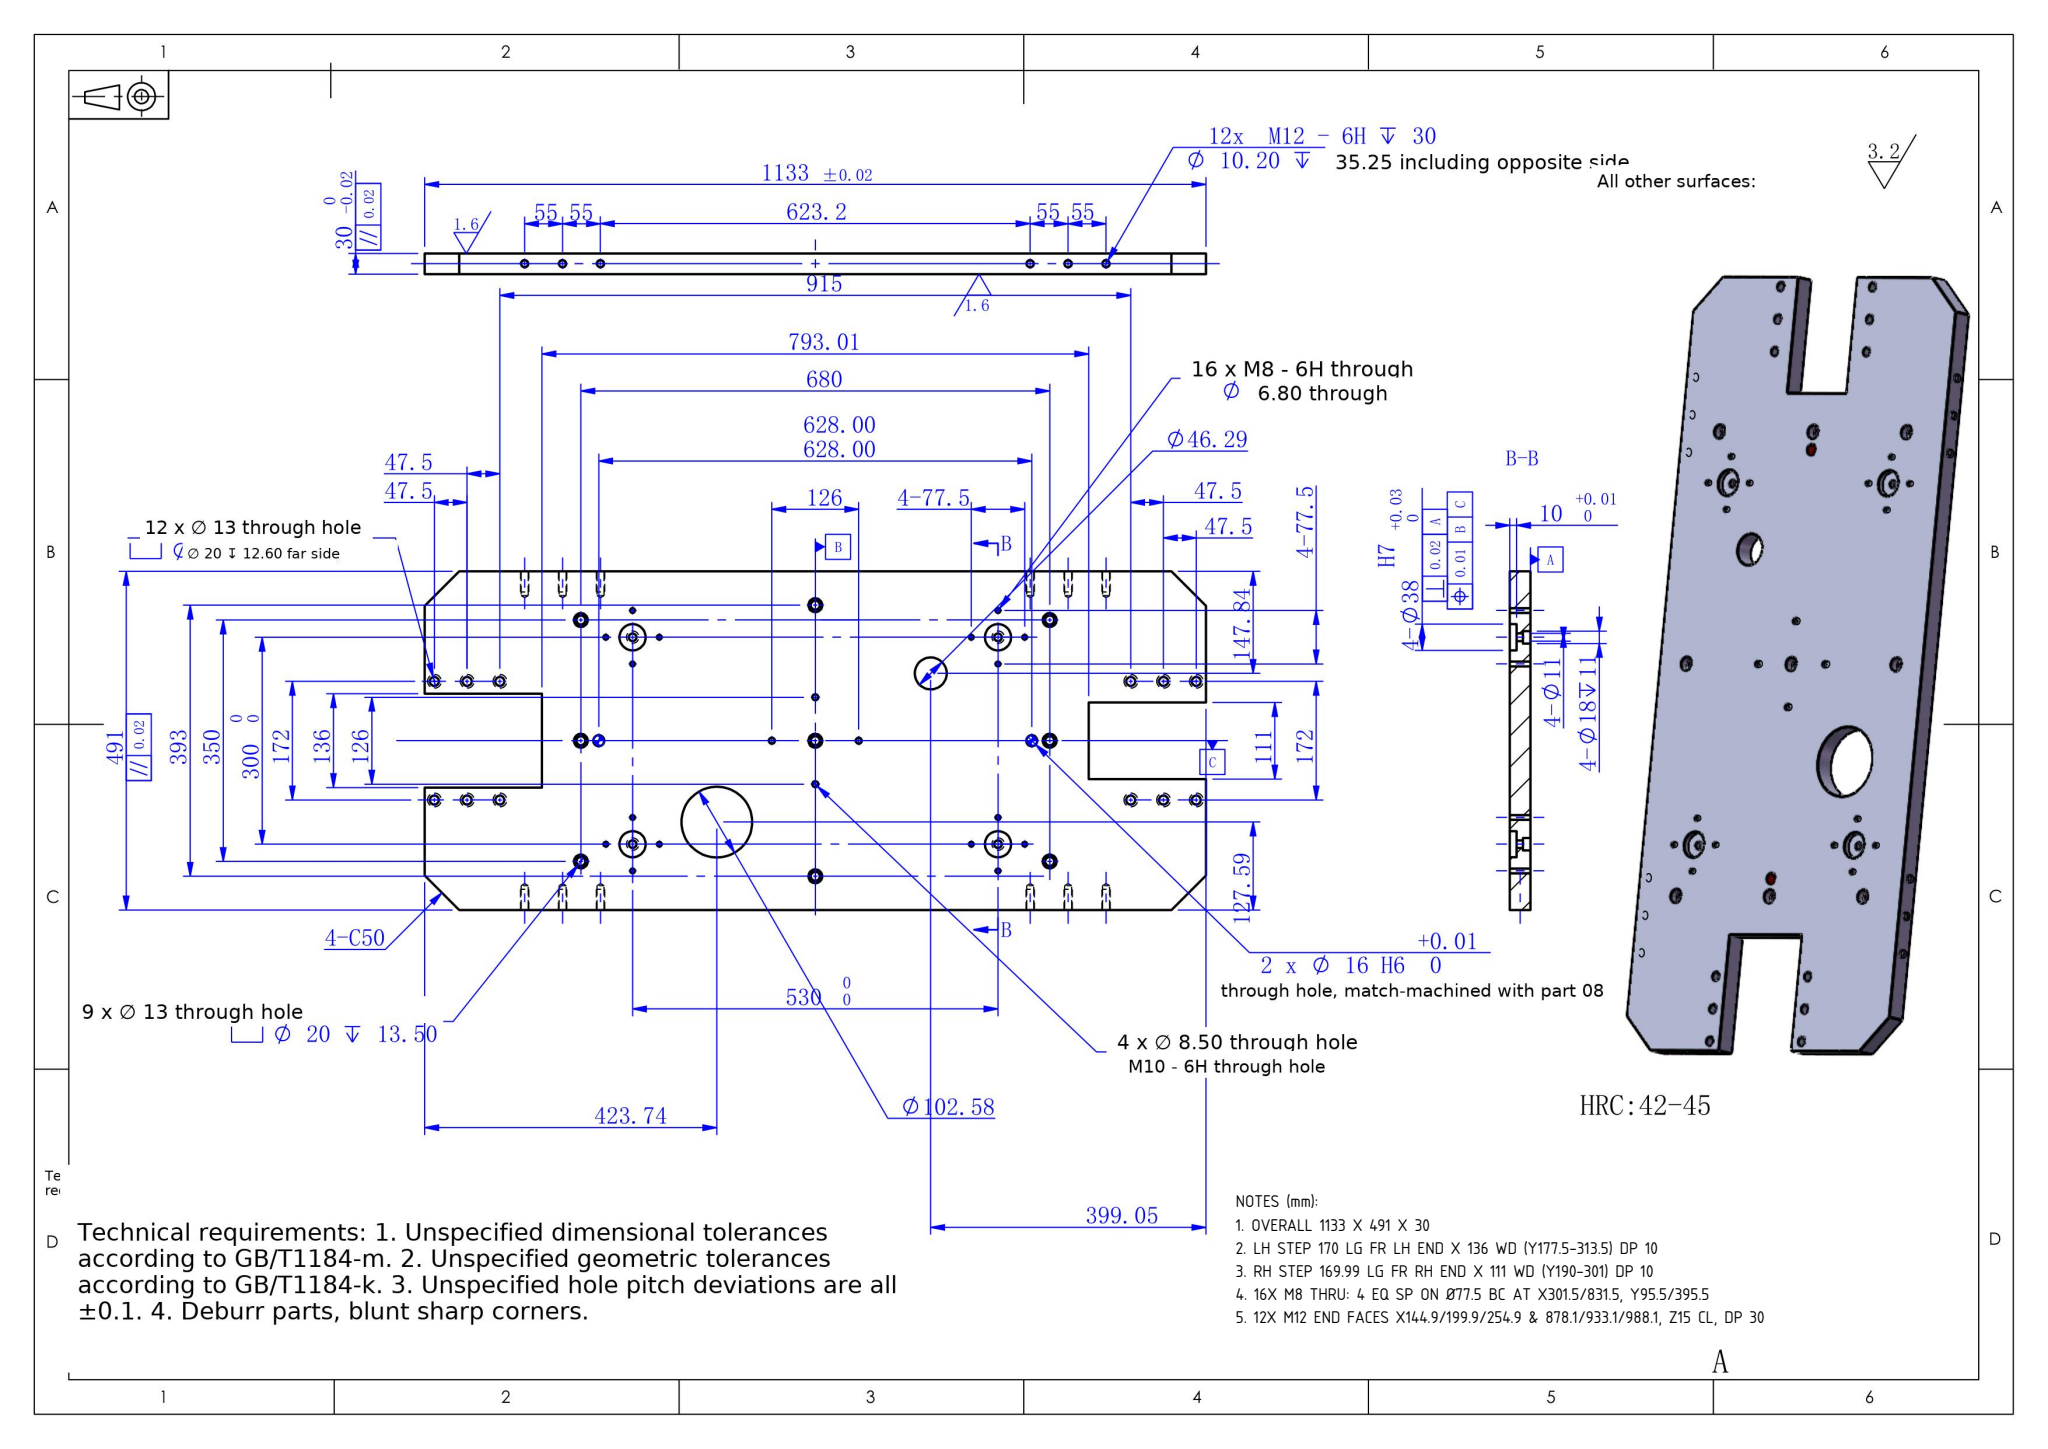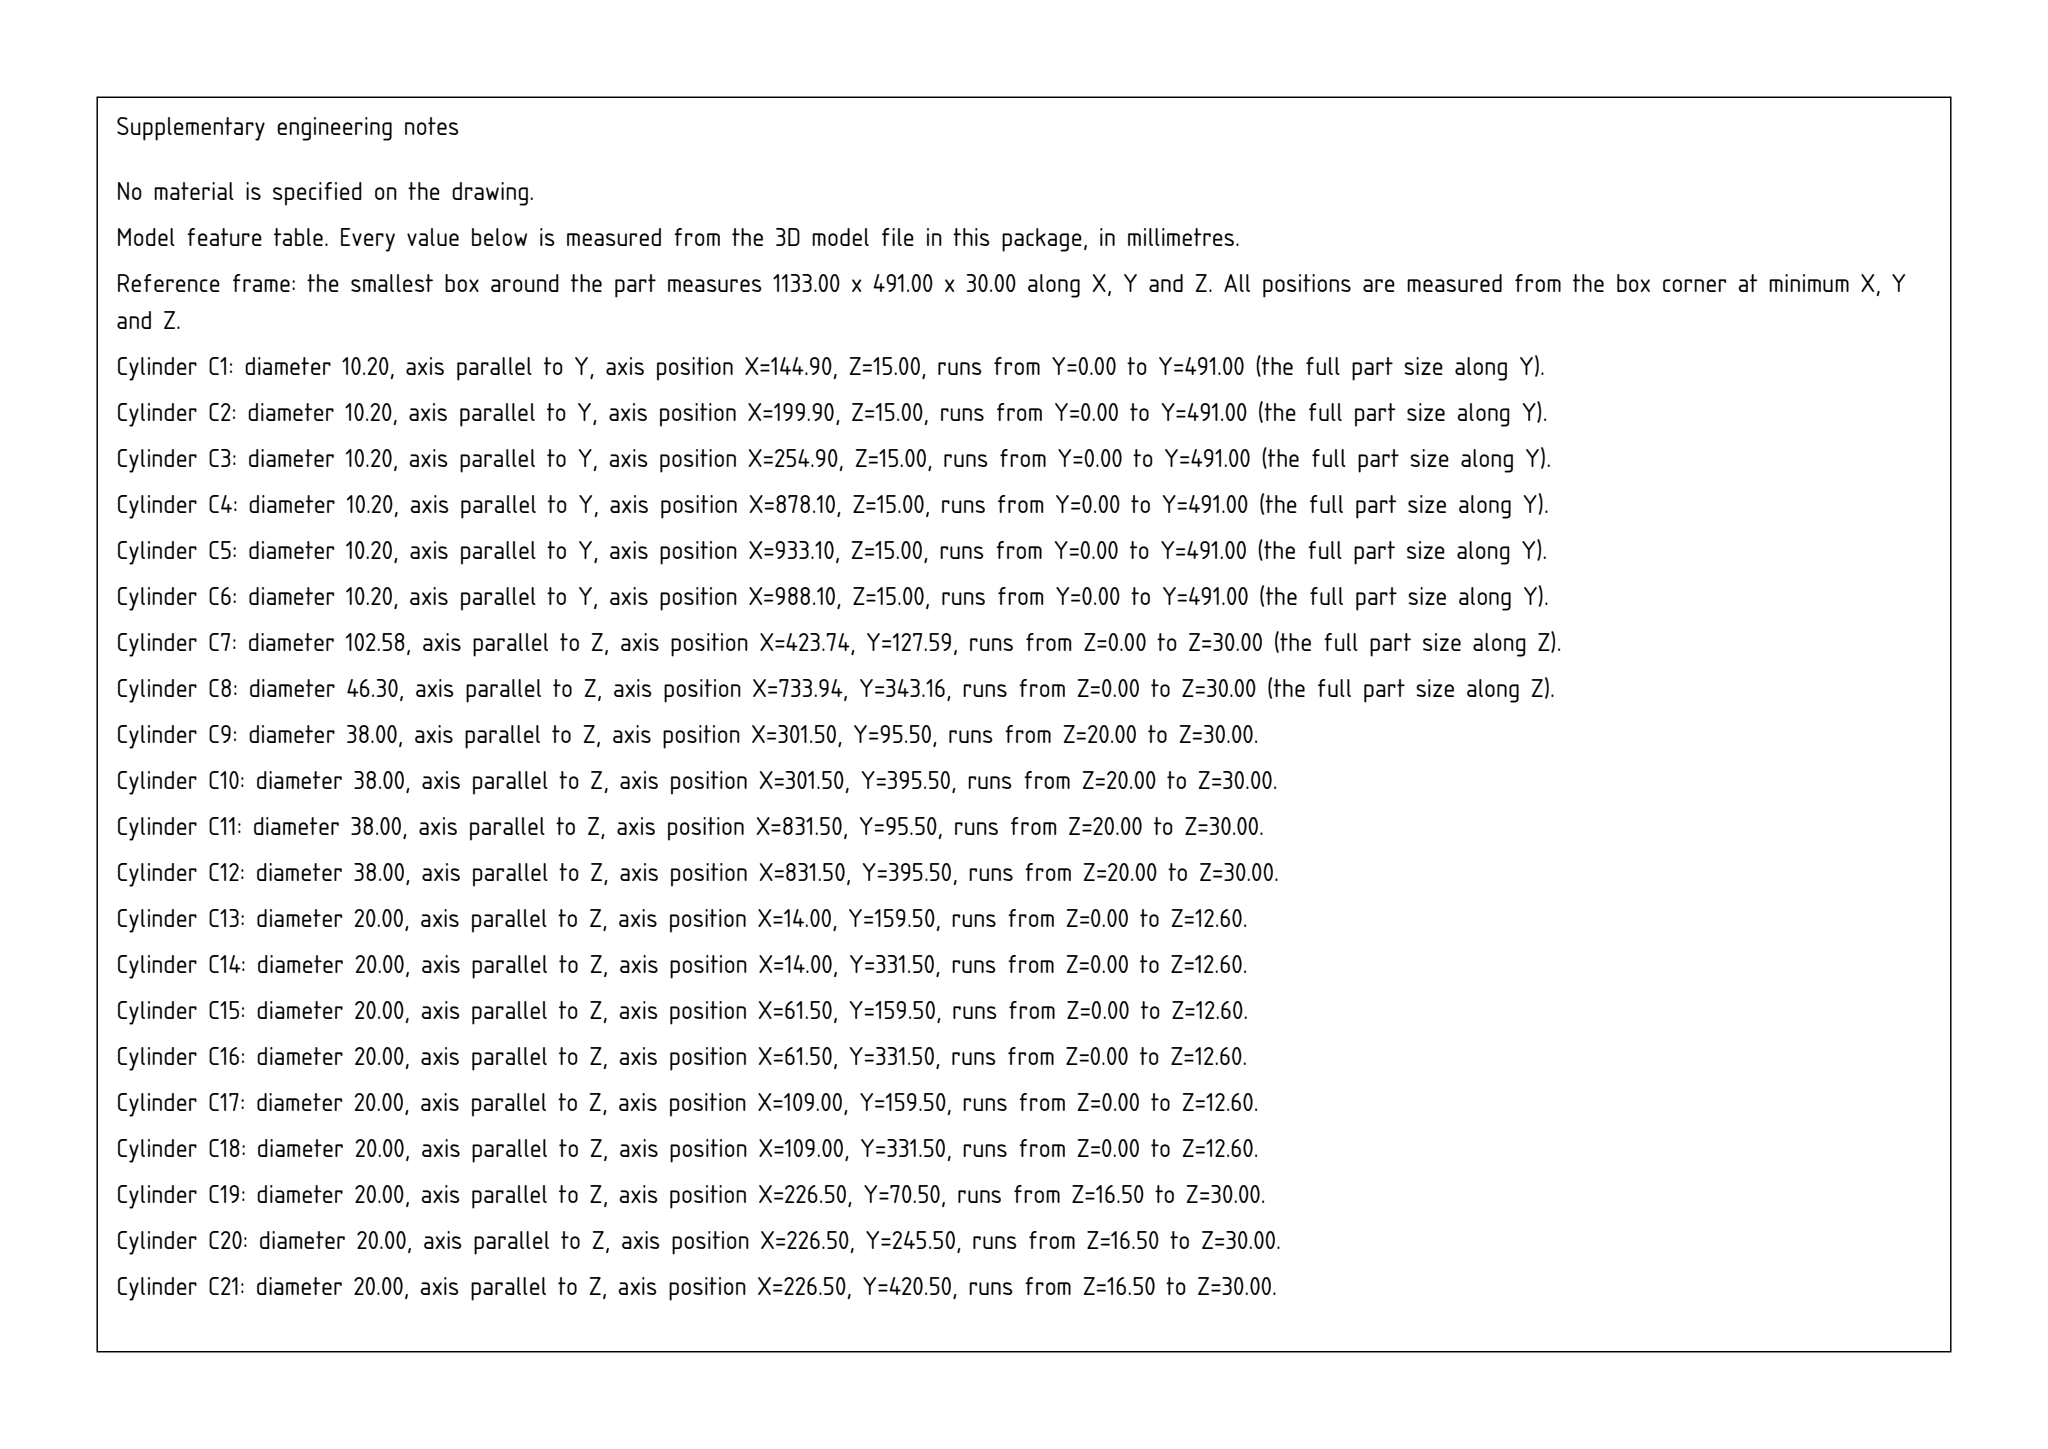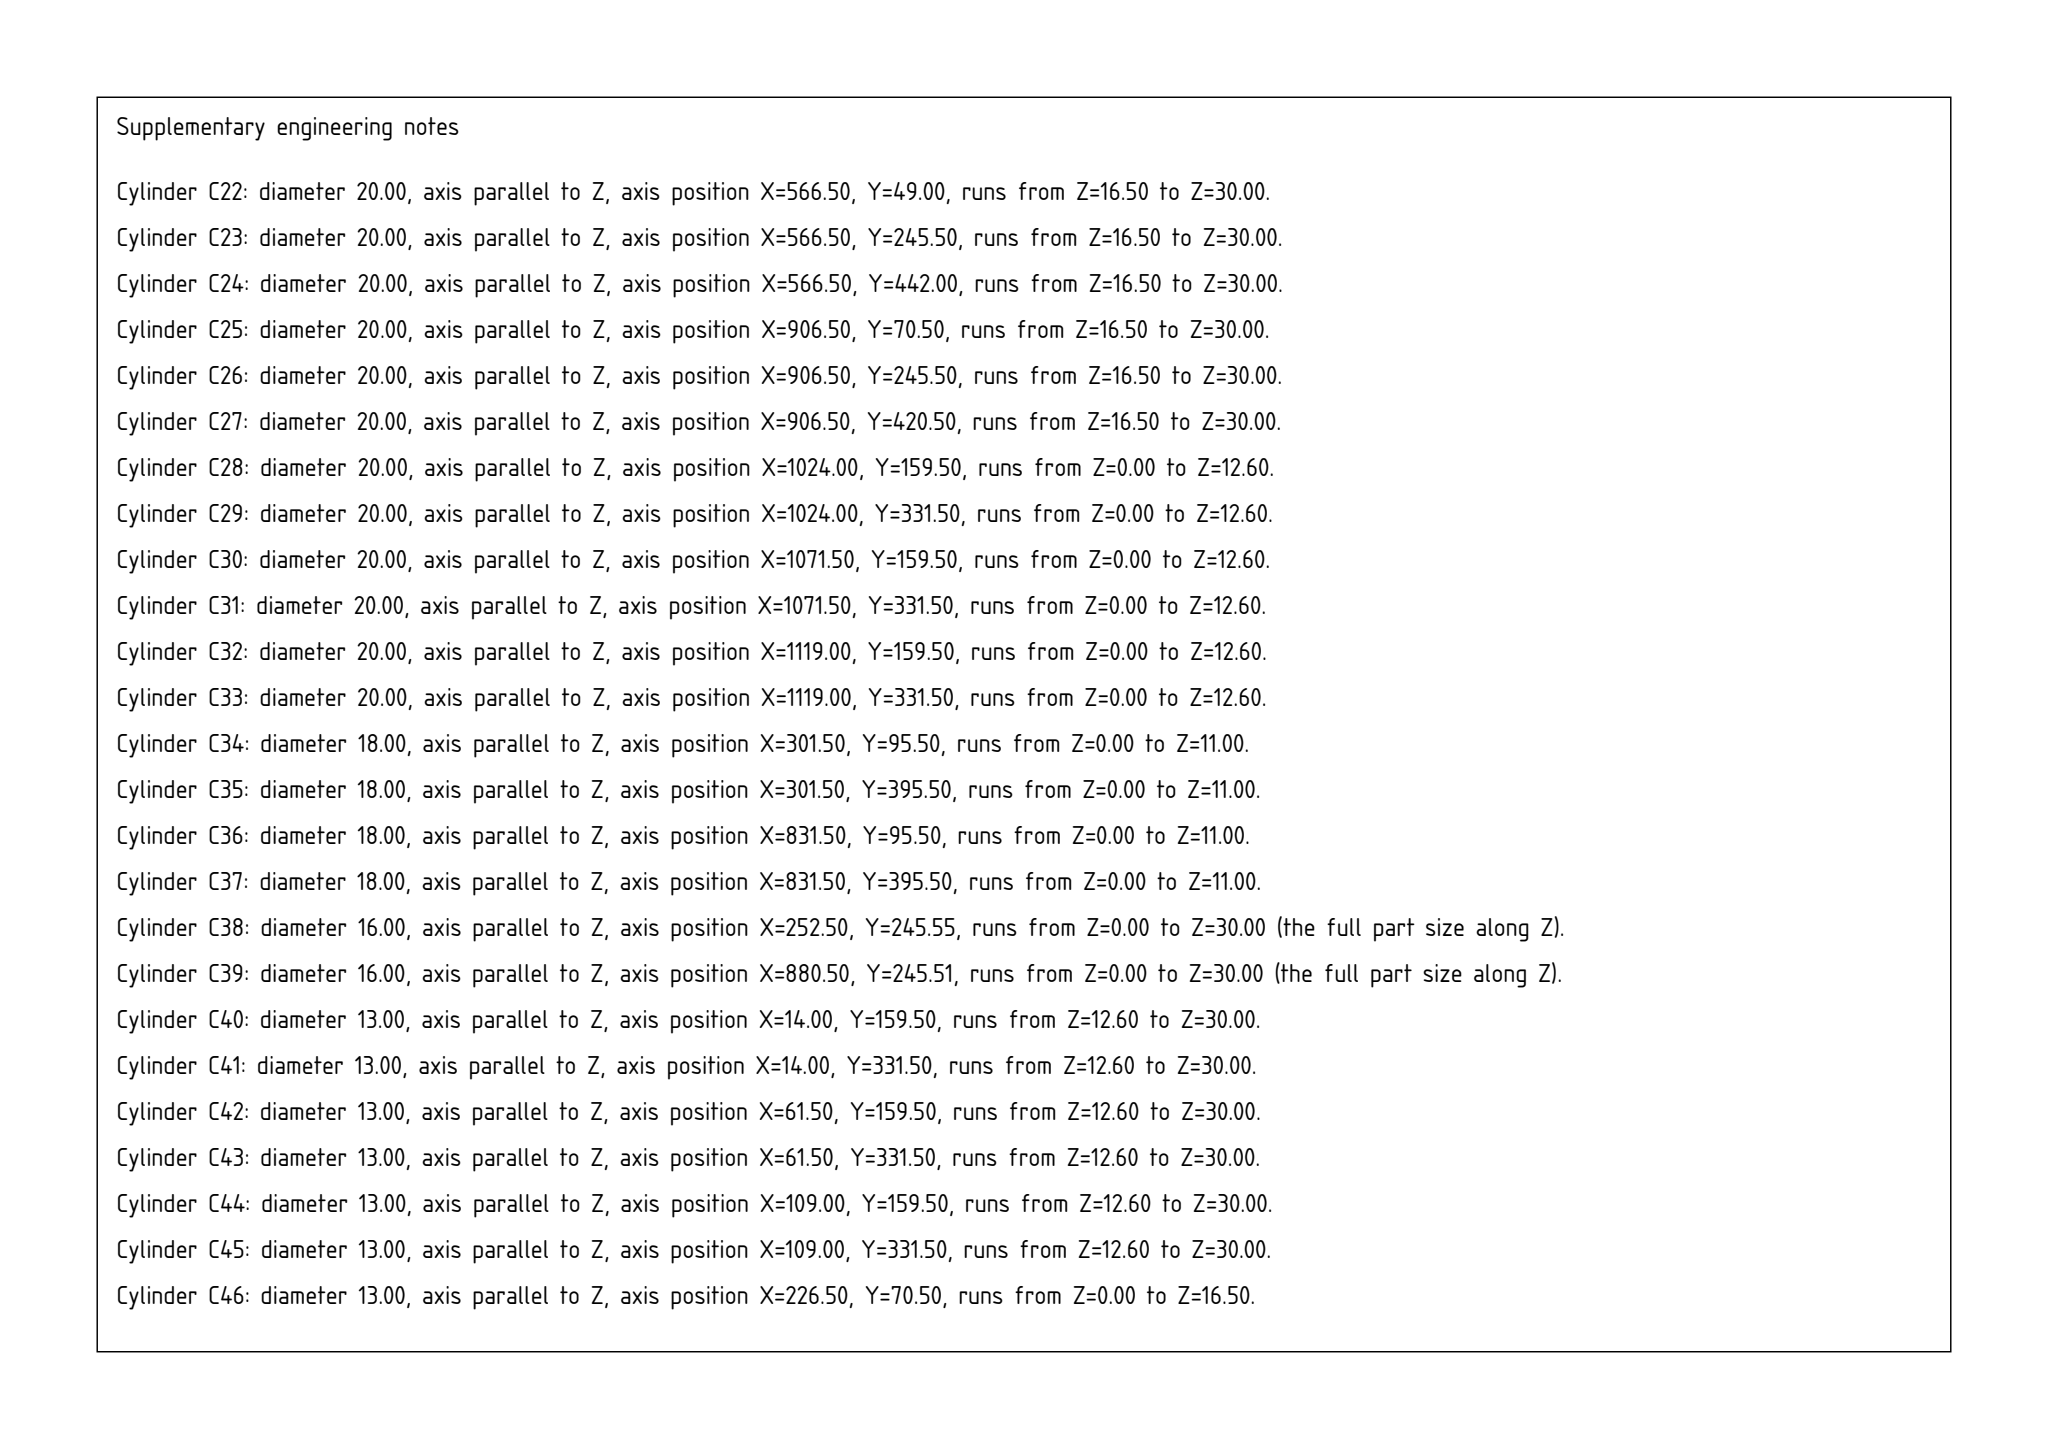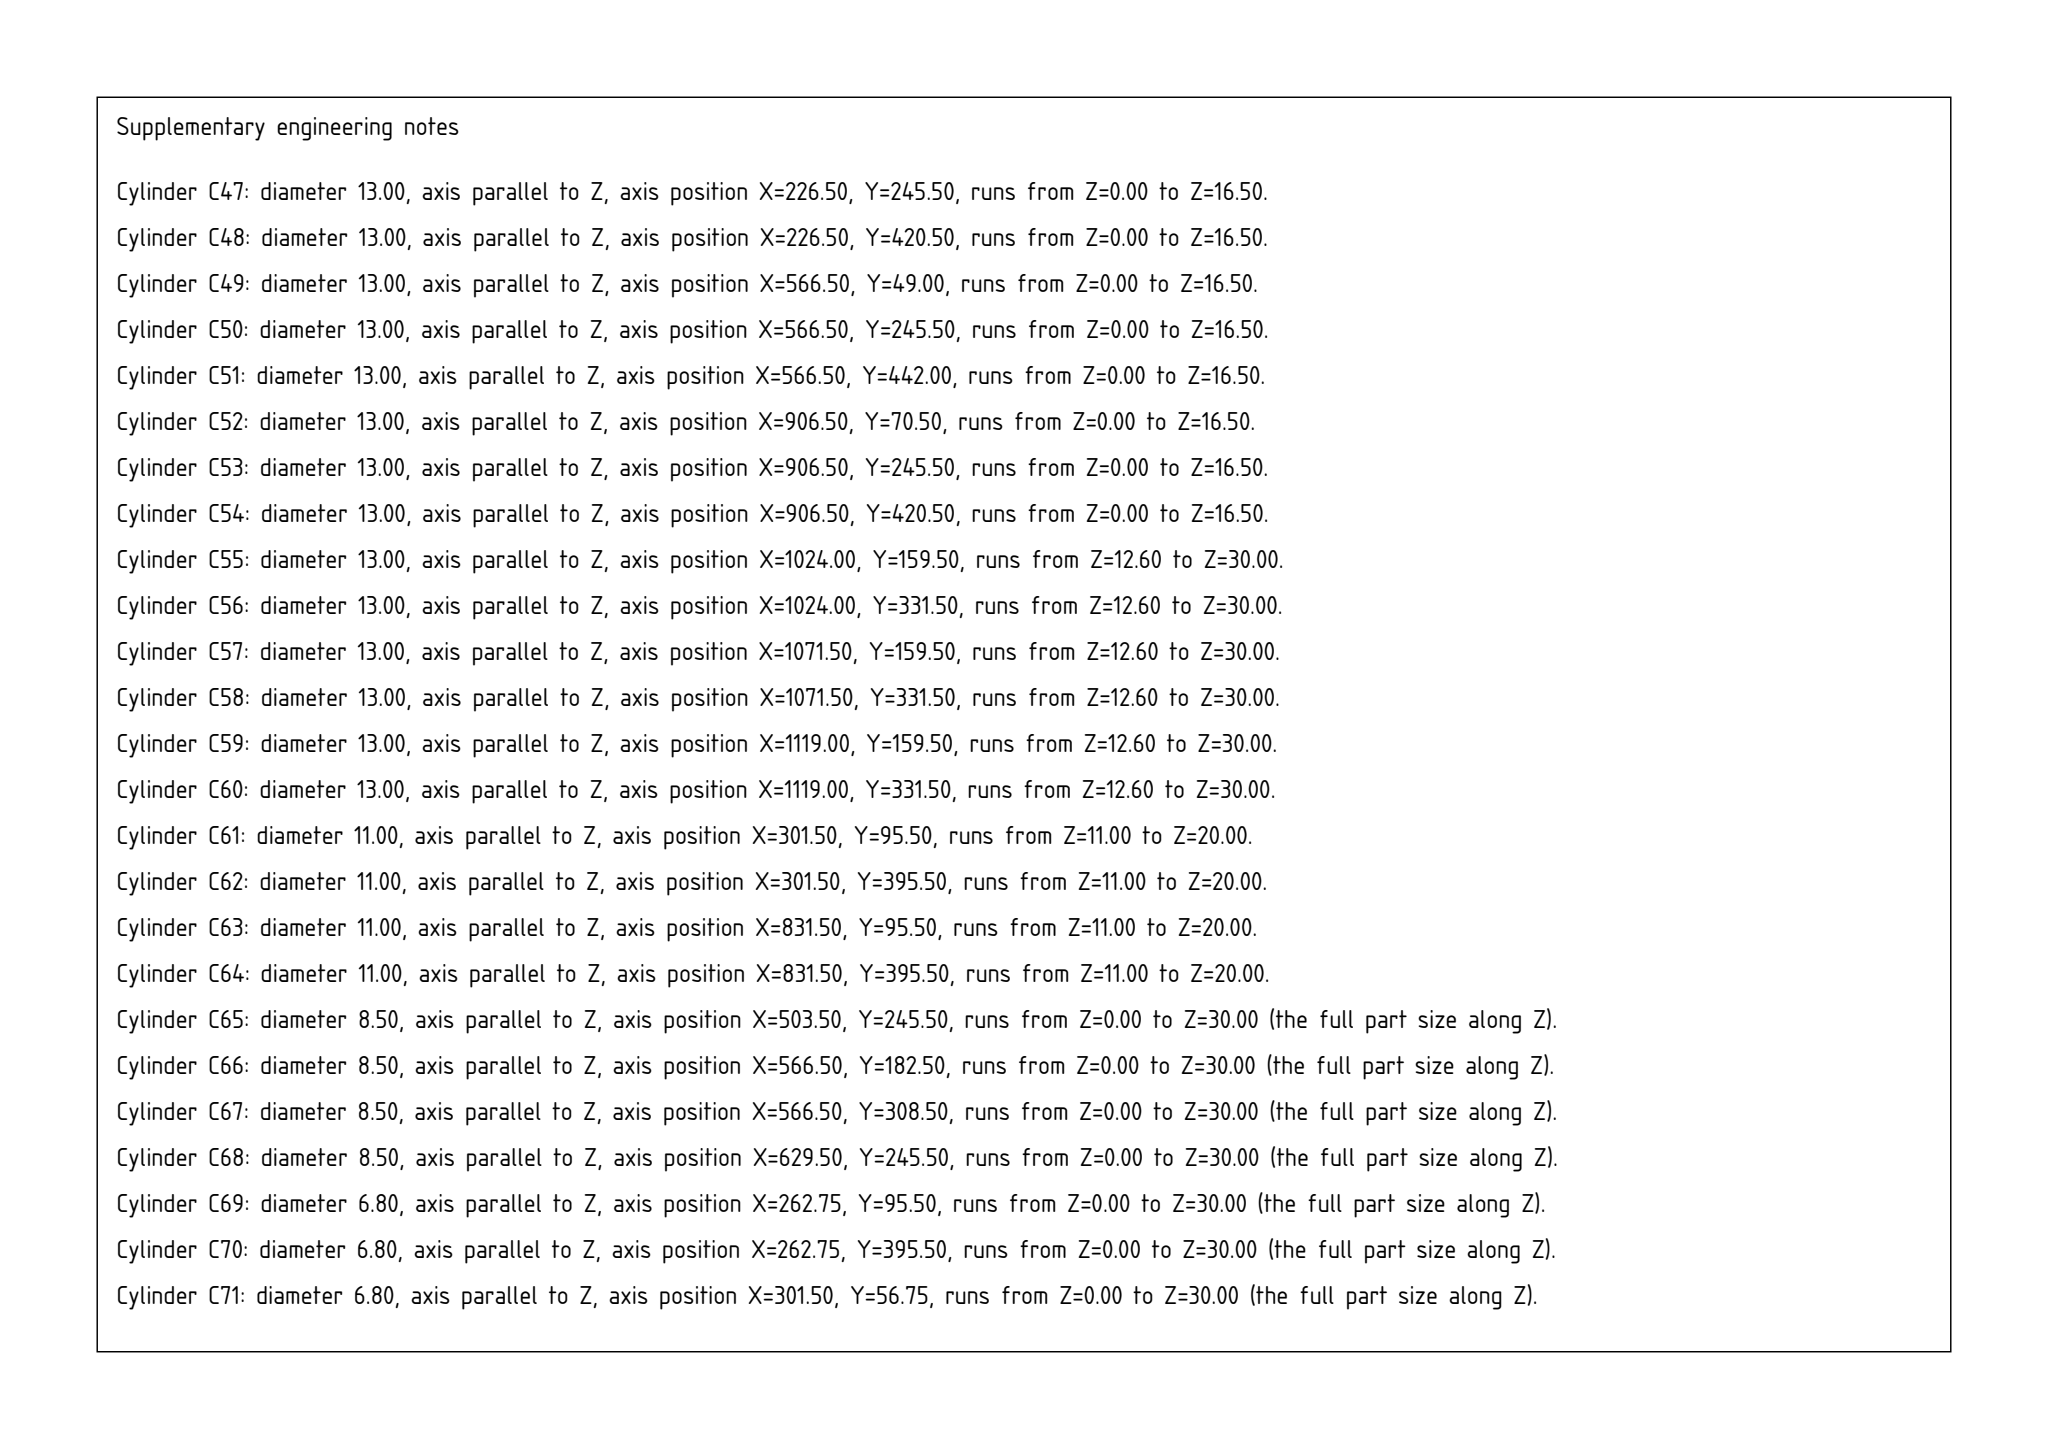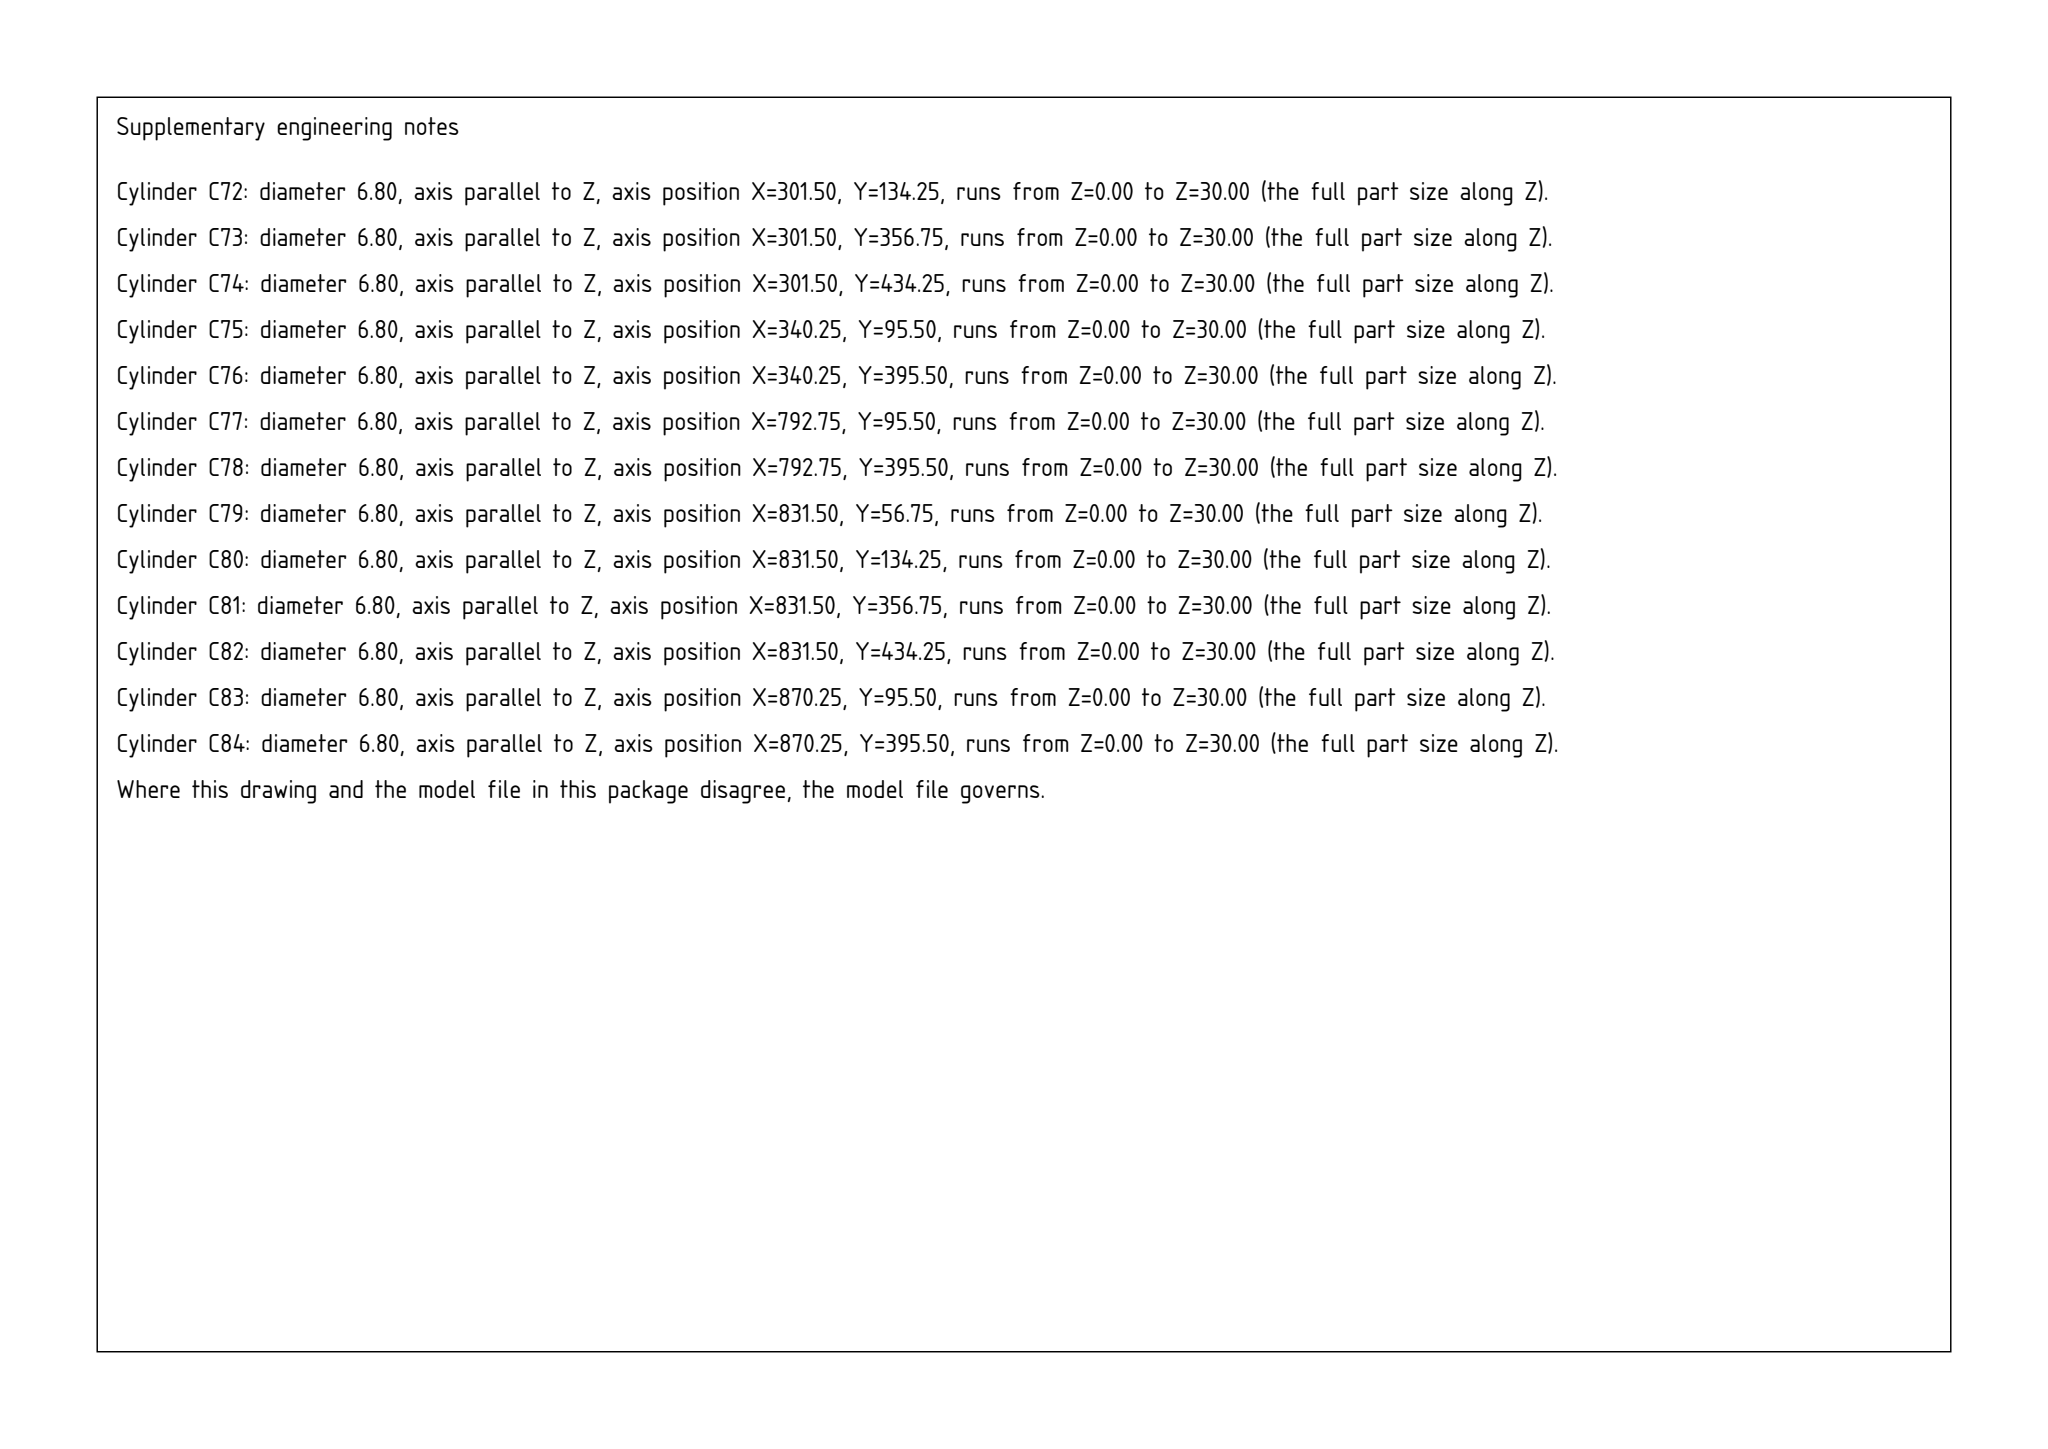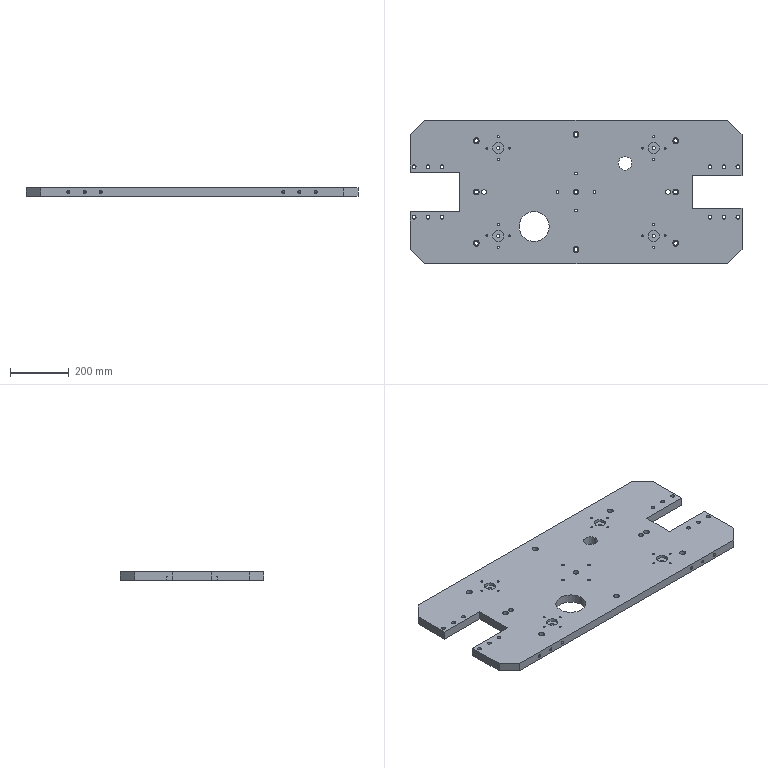Part | SolidWorks | mm | 1 solid | 251 faces | box 1133 x 491 x 30 mm | volume 14716018 mm3 | cylinder 180 | plane 47 | cone 24 | commonest cylinder face diameters 20 x42 13 x42 6.8 x32 10.2 x24 18 x8 11 x8 38 x8 8.5 x8
Drawing notes:
OVERALL 1133 X 491 X 30 | from the solid: bbox_xyz [1133.0, 491.0, 30.0]
LH STEP 170 LG FR LH END X 136 WD (Y177.5-313.5) DP 10 | from the solid: x plane 170.0; y planes 177.5 & 313.5; z plane 20.0 (30-20=10 deep)
RH STEP 169.99 LG FR RH END X 111 WD (Y190-301) DP 10 | from the solid: x plane 963.01 (1133-963.01); y planes 190.0 & 301.0; z plane 20.0
16X M8 THRU: 4 EQ SP ON Ø77.5 BC AT X301.5/831.5, Y95.5/395.5 | from the solid: Ø6.8 z-holes at (262.75/340.25, 95.5 & 395.5) and (301.5, 56.75/134.25) etc.; 38.75 offset = Ø77.5 BC
12X M12 END FACES X144.9/199.9/254.9 & 878.1/933.1/988.1, Z15 CL, DP 30 | from the solid: Ø10.2 y-axis holes at those x, z=15.0, length 35.25, pitch 55, plate thk 30
build123d program:
from build123d import *

# Parameters (mm, degrees)
SKETCH1_W                                        = 1133
SKETCH1_H                                        = 491
BOSS_EXTRUDE1_DEPTH                              = 30
SKETCH2_W                                        = 169.999
SKETCH2_H                                        = 111
CUT_EXTRUDE1_DEPTH                               = 5130.375
SKETCH3_W                                        = 170
SKETCH3_H                                        = 136
CUT_EXTRUDE2_DEPTH                               = 5130.375
M12_HEX_SOCKET_HEAD_CAP_SCREW_CBORE1_D           = 13
M12_HEX_SOCKET_HEAD_CAP_SCREW_CBORE1_CBORE_D     = 20
M12_HEX_SOCKET_HEAD_CAP_SCREW_CBORE1_CBORE_DEPTH = 12.6
M12_TAPPED_HOLE1_AT_2_COUNT                      = 2
M12_TAPPED_HOLE1_AT_2_PITCH                      = 55
M12_TAPPED_HOLE1_AT_3_COUNT                      = 2
M12_TAPPED_HOLE1_AT_3_PITCH                      = 110
M12_TAPPED_HOLE1_AT_4_COUNT                      = 2
M12_TAPPED_HOLE1_AT_4_PITCH                      = 623.2
M12_TAPPED_HOLE1_AT_5_COUNT                      = 2
M12_TAPPED_HOLE1_AT_5_PITCH                      = 678.2
M12_TAPPED_HOLE1_AT_6_COUNT                      = 2
M12_TAPPED_HOLE1_AT_6_PITCH                      = 733.2
CHAMFER1_SIZE                                    = 50
M10_TAPPED_HOLE1_D                               = 8.5
M12_HEX_HEAD_BOLT_COUNTERBORE_1_D                = 13
M12_HEX_HEAD_BOLT_COUNTERBORE_1_CBORE_D          = 20
M12_HEX_HEAD_BOLT_COUNTERBORE_1_CBORE_DEPTH      = 13.5
SKETCH19_R                                       = 19
CUT_EXTRUDE3_DEPTH                               = 10
M10_HEX_HEAD_BOLT_COUNTERBORE_1_D                = 11
M10_HEX_HEAD_BOLT_COUNTERBORE_1_CBORE_D          = 18
M10_HEX_HEAD_BOLT_COUNTERBORE_1_CBORE_DEPTH      = 11
M8_TAPPED_HOLE1_D                                = 6.8
MIRROR4_COPY_1_SKETCH_R                          = 19
MIRROR4_COPY_1_DEPTH                             = 10
MIRROR4_COPY_2_D                                 = 11
MIRROR4_COPY_2_CBORE_D                           = 18
MIRROR4_COPY_2_CBORE_DEPTH                       = 11
MIRROR4_COPY_3_D                                 = 6.8
F_16_0_16_DIAMETER_HOLE1_D                       = 16
SKETCH26_R                                       = 23.147
SKETCH26_R_2                                     = 51.292
CUT_EXTRUDE4_DEPTH                               = 359


with BuildPart() as part:
    # Sketch1 → Boss-Extrude1 (new body)
    with BuildSketch(Plane.XY.offset(289.6)):
        with Locations((-3796.515, -2451.478)):
            Rectangle(SKETCH1_W, SKETCH1_H)
    extrude(amount=-BOSS_EXTRUDE1_DEPTH)

    # Sketch2 → Cut-Extrude1 (cut, through all)
    with BuildSketch(Plane(origin=(0, 0, 259.6), x_dir=(-1, 0, 0), z_dir=(0, 0, -1))):
        with Locations((3315.005, -2451.478)):
            Rectangle(SKETCH2_W, SKETCH2_H)
    extrude(amount=-CUT_EXTRUDE1_DEPTH, mode=Mode.SUBTRACT)

    # Sketch3 → Cut-Extrude2 (cut, through all)
    with BuildSketch(Plane(origin=(0, 0, 259.6), x_dir=(-1, 0, 0), z_dir=(0, 0, -1))):
        with Locations((4278.015, -2451.478)):
            Rectangle(SKETCH3_W, SKETCH3_H)
    extrude(amount=-CUT_EXTRUDE2_DEPTH, mode=Mode.SUBTRACT)

    # M12 Hex Socket Head Cap Screw CBORE1 (through all)
    with Locations(Plane(origin=(0, 0, 259.6), x_dir=(-1, 0, 0), z_dir=(0, 0, -1))):
        with Locations((4349.015, -2365.478), (4301.515, -2365.478), (4254.015, -2365.478), (4254.015, -2537.478), (4301.515, -2537.478), (4349.015, -2537.478)):
            m12_hex_socket_head_cap_screw_cbore1 = CounterBoreHole(M12_HEX_SOCKET_HEAD_CAP_SCREW_CBORE1_D / 2, M12_HEX_SOCKET_HEAD_CAP_SCREW_CBORE1_CBORE_D / 2, M12_HEX_SOCKET_HEAD_CAP_SCREW_CBORE1_CBORE_DEPTH)

    # Mirror1: M12 Hex Socket Head Cap Screw CBORE1 across plane
    add(m12_hex_socket_head_cap_screw_cbore1.mirror(Plane.ZY.offset(3796.515)), mode=Mode.SUBTRACT)

    # Sketch6 → M12 Tapped Hole1 (revolve, cut)
    with BuildSketch(Plane(origin=(-4108.115, -2696.978, 274.6), x_dir=(0, 0, -1), z_dir=(1, 0, 0))):
        Polygon((0, 0), (0, 38.314), (5.1, 35.25), (5.1, 0), align=None)
    m12_tapped_hole1 = revolve(axis=Axis((-4108.115, -2703.328, 274.6), (0, 1, 0)), mode=Mode.SUBTRACT)

    # M12 Tapped Hole1 at 2: M12 Tapped Hole1 ×2
    with Locations(*[(-i * M12_TAPPED_HOLE1_AT_2_PITCH, 0, 0) for i in range(1, M12_TAPPED_HOLE1_AT_2_COUNT)]):
        add(m12_tapped_hole1, mode=Mode.SUBTRACT)

    # M12 Tapped Hole1 at 3: M12 Tapped Hole1 ×2
    with Locations(*[(-i * M12_TAPPED_HOLE1_AT_3_PITCH, 0, 0) for i in range(1, M12_TAPPED_HOLE1_AT_3_COUNT)]):
        add(m12_tapped_hole1, mode=Mode.SUBTRACT)

    # M12 Tapped Hole1 at 4: M12 Tapped Hole1 ×2
    with Locations(*[(i * M12_TAPPED_HOLE1_AT_4_PITCH, 0, 0) for i in range(1, M12_TAPPED_HOLE1_AT_4_COUNT)]):
        add(m12_tapped_hole1, mode=Mode.SUBTRACT)

    # M12 Tapped Hole1 at 5: M12 Tapped Hole1 ×2
    with Locations(*[(i * M12_TAPPED_HOLE1_AT_5_PITCH, 0, 0) for i in range(1, M12_TAPPED_HOLE1_AT_5_COUNT)]):
        add(m12_tapped_hole1, mode=Mode.SUBTRACT)

    # M12 Tapped Hole1 at 6: M12 Tapped Hole1 ×2
    with Locations(*[(i * M12_TAPPED_HOLE1_AT_6_PITCH, 0, 0) for i in range(1, M12_TAPPED_HOLE1_AT_6_COUNT)]):
        add(m12_tapped_hole1, mode=Mode.SUBTRACT)

    # Mirror2: M12 Tapped Hole1 across plane
    add(m12_tapped_hole1.mirror(Plane(origin=(0, -2451.478, 0), x_dir=(0, 0, 1), z_dir=(0, -1, 0))), mode=Mode.SUBTRACT)

    # Mirror2 copy 1 sketch → Mirror2 copy 1 (revolve, cut)
    with BuildSketch(Plane(origin=(-4163.115, -2205.978, 274.6), x_dir=(0, 0, -1), z_dir=(1, 0, 0))):
        Polygon((0, 0), (0, -38.314), (5.1, -35.25), (5.1, 0), align=None)
    revolve(axis=Axis((-4163.115, -2199.628, 274.6), (0, 1, 0)), mode=Mode.SUBTRACT)

    # Mirror2 copy 2 sketch → Mirror2 copy 2 (revolve, cut)
    with BuildSketch(Plane(origin=(-4218.115, -2205.978, 274.6), x_dir=(0, 0, -1), z_dir=(1, 0, 0))):
        Polygon((0, 0), (0, -38.314), (5.1, -35.25), (5.1, 0), align=None)
    revolve(axis=Axis((-4218.115, -2199.628, 274.6), (0, 1, 0)), mode=Mode.SUBTRACT)

    # Mirror2 copy 3 sketch → Mirror2 copy 3 (revolve, cut)
    with BuildSketch(Plane(origin=(-3484.915, -2205.978, 274.6), x_dir=(0, 0, -1), z_dir=(1, 0, 0))):
        Polygon((0, 0), (0, -38.314), (5.1, -35.25), (5.1, 0), align=None)
    revolve(axis=Axis((-3484.915, -2199.628, 274.6), (0, 1, 0)), mode=Mode.SUBTRACT)

    # Mirror2 copy 4 sketch → Mirror2 copy 4 (revolve, cut)
    with BuildSketch(Plane(origin=(-3429.915, -2205.978, 274.6), x_dir=(0, 0, -1), z_dir=(1, 0, 0))):
        Polygon((0, 0), (0, -38.314), (5.1, -35.25), (5.1, 0), align=None)
    revolve(axis=Axis((-3429.915, -2199.628, 274.6), (0, 1, 0)), mode=Mode.SUBTRACT)

    # Mirror2 copy 5 sketch → Mirror2 copy 5 (revolve, cut)
    with BuildSketch(Plane(origin=(-3374.915, -2205.978, 274.6), x_dir=(0, 0, -1), z_dir=(1, 0, 0))):
        Polygon((0, 0), (0, -38.314), (5.1, -35.25), (5.1, 0), align=None)
    revolve(axis=Axis((-3374.915, -2199.628, 274.6), (0, 1, 0)), mode=Mode.SUBTRACT)

    # Chamfer1
    chamfer1_edges = [part.edges().sort_by_distance(p)[0] for p in [
        (-4363.015, -2696.978, 274.6),
        (-4363.015, -2205.978, 274.6),
        (-3230.015, -2205.978, 274.6),
        (-3230.015, -2696.978, 274.6),
    ]]
    chamfer(chamfer1_edges, length=CHAMFER1_SIZE)

    # M10 Tapped Hole1 (through all)
    with Locations(Plane.XY.offset(289.6)):
        with Locations((-3796.515, -2388.478), (-3733.515, -2451.478), (-3796.515, -2514.478), (-3859.515, -2451.478)):
            Hole(M10_TAPPED_HOLE1_D / 2)

    # M12 Hex Head Bolt Counterbore 1 (through all)
    with Locations(Plane.XY.offset(289.6)):
        with Locations((-3456.515, -2451.478), (-3796.515, -2451.478), (-4136.515, -2451.478), (-3456.515, -2626.478), (-3796.515, -2647.978), (-4136.515, -2626.478), (-3796.515, -2254.978), (-3456.515, -2276.478), (-4136.515, -2276.478)):
            CounterBoreHole(M12_HEX_HEAD_BOLT_COUNTERBORE_1_D / 2, M12_HEX_HEAD_BOLT_COUNTERBORE_1_CBORE_D / 2, M12_HEX_HEAD_BOLT_COUNTERBORE_1_CBORE_DEPTH)

    # Sketch19 → Cut-Extrude3 (cut)
    with BuildSketch(Plane.XY.offset(289.6)):
        with Locations((-4061.515, -2601.478)):
            Circle(SKETCH19_R)
    cut_extrude3 = extrude(amount=-CUT_EXTRUDE3_DEPTH, mode=Mode.SUBTRACT)

    # M10 Hex Head Bolt Counterbore 1 (through all)
    with Locations(Plane(origin=(0, 0, 259.6), x_dir=(-1, 0, 0), z_dir=(0, 0, -1))):
        with Locations((4061.515, -2601.478)):
            m10_hex_head_bolt_counterbore_1 = CounterBoreHole(M10_HEX_HEAD_BOLT_COUNTERBORE_1_D / 2, M10_HEX_HEAD_BOLT_COUNTERBORE_1_CBORE_D / 2, M10_HEX_HEAD_BOLT_COUNTERBORE_1_CBORE_DEPTH)

    # M8 Tapped Hole1 (through all)
    with Locations(Plane.XY.offset(289.6)):
        with Locations((-4100.265, -2601.478), (-4061.515, -2562.728), (-4022.765, -2601.478), (-4061.515, -2640.228)):
            m8_tapped_hole1 = Hole(M8_TAPPED_HOLE1_D / 2)

    # Mirror3: Cut-Extrude3, M10 Hex Head Bolt Counterbore 1, M8 Tapped Hole1 across plane
    add(cut_extrude3.mirror(Plane(origin=(0, -2451.478, 0), x_dir=(0, 0, 1), z_dir=(0, -1, 0))), mode=Mode.SUBTRACT)
    add(m10_hex_head_bolt_counterbore_1.mirror(Plane(origin=(0, -2451.478, 0), x_dir=(0, 0, 1), z_dir=(0, -1, 0))), mode=Mode.SUBTRACT)
    add(m8_tapped_hole1.mirror(Plane(origin=(0, -2451.478, 0), x_dir=(0, 0, 1), z_dir=(0, -1, 0))), mode=Mode.SUBTRACT)

    # Mirror4: Cut-Extrude3, M10 Hex Head Bolt Counterbore 1, M8 Tapped Hole1 across plane
    add(cut_extrude3.mirror(Plane.ZY.offset(3796.515)), mode=Mode.SUBTRACT)
    add(m10_hex_head_bolt_counterbore_1.mirror(Plane.ZY.offset(3796.515)), mode=Mode.SUBTRACT)
    add(m8_tapped_hole1.mirror(Plane.ZY.offset(3796.515)), mode=Mode.SUBTRACT)

    # Mirror4 copy 1 sketch → Mirror4 copy 1 (cut)
    with BuildSketch(Plane(origin=(-7593.03, -4902.957, 289.6), x_dir=(-1, 0, 0), z_dir=(0, 0, 1))):
        with Locations((-4061.515, -2601.478)):
            Circle(MIRROR4_COPY_1_SKETCH_R)
    extrude(amount=-MIRROR4_COPY_1_DEPTH, mode=Mode.SUBTRACT)

    # Mirror4 copy 2 (through all)
    with Locations(Plane(origin=(-7593.03, -4902.957, 259.6), x_dir=(1, 0, 0), z_dir=(0, 0, -1))):
        with Locations((4061.515, -2601.478)):
            CounterBoreHole(MIRROR4_COPY_2_D / 2, MIRROR4_COPY_2_CBORE_D / 2, MIRROR4_COPY_2_CBORE_DEPTH)

    # Mirror4 copy 3 (through all)
    with Locations(Plane(origin=(-7593.03, -4902.957, 289.6), x_dir=(-1, 0, 0), z_dir=(0, 0, 1))):
        with Locations((-4100.265, -2601.478), (-4061.515, -2562.728), (-4022.765, -2601.478), (-4061.515, -2640.228)):
            Hole(MIRROR4_COPY_3_D / 2)

    # 16.0 _16_ Diameter Hole1 (through all)
    with Locations(Plane(origin=(0, 0, 259.6), x_dir=(-1, 0, 0), z_dir=(0, 0, -1))):
        with Locations((4110.515, -2451.433), (3482.515, -2451.474)):
            Hole(F_16_0_16_DIAMETER_HOLE1_D / 2)

    # Sketch26 → Cut-Extrude4 (cut)
    with BuildSketch(Plane(origin=(0, 0, 259.6), x_dir=(-1, 0, 0), z_dir=(0, 0, -1))):
        with Locations((3629.069, -2353.822)):
            Circle(SKETCH26_R)
        with Locations((3939.274, -2569.388)):
            Circle(SKETCH26_R_2)
    extrude(amount=-CUT_EXTRUDE4_DEPTH, mode=Mode.SUBTRACT)


solid = part.part